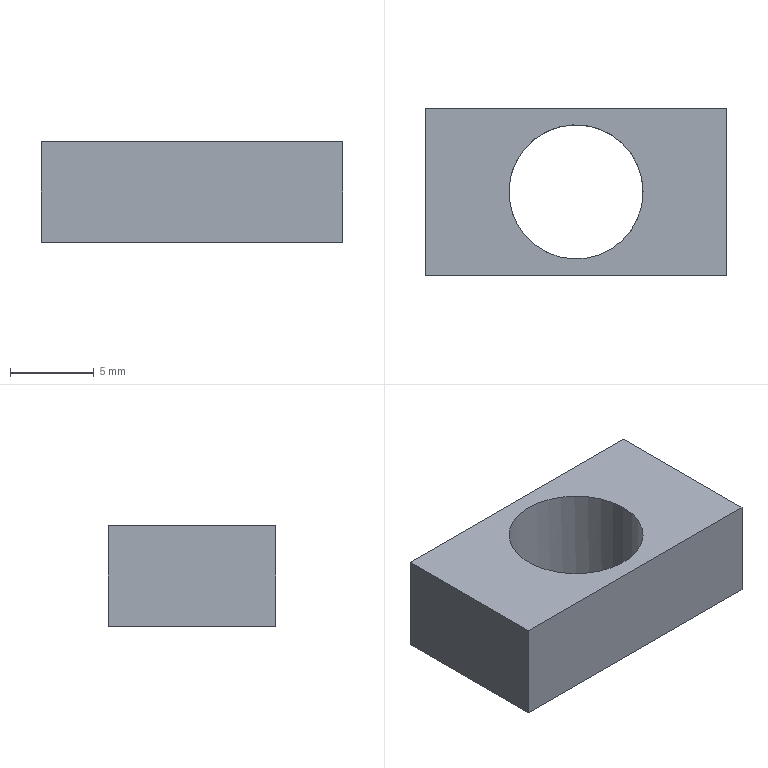Component | NX | WORKPIECE_PROCESSED | 1 solid | 7 faces | box 18 x 10 x 6 mm | volume 778 mm3 | plane 6 | cylinder 1 | commonest cylinder face diameters 8 x1
STEP:
#1=CARTESIAN_POINT('',(0.,0.,0.));
#2=DIRECTION('',(0.,0.,1.));
#3=DIRECTION('',(1.,0.,0.));
#4=AXIS2_PLACEMENT_3D('',#1,#2,#3);
#5=CARTESIAN_POINT('',(-142.329,14.498,29.));
#6=VERTEX_POINT('',#5);
#7=CARTESIAN_POINT('',(-146.329,14.498,29.));
#8=DIRECTION('',(0.,0.,1.));
#9=DIRECTION('',(1.,0.,0.));
#10=AXIS2_PLACEMENT_3D('',#7,#8,#9);
#11=CIRCLE('',#10,4.);
#12=CARTESIAN_POINT('',(-146.329,14.498,29.));
#13=DIRECTION('',(0.,0.,1.));
#14=DIRECTION('',(1.,0.,0.));
#15=AXIS2_PLACEMENT_3D('',#12,#13,#14);
#16=PLANE('',#15);
#17=CARTESIAN_POINT('',(0.,0.));
#18=DIRECTION('',(1.,0.));
#19=AXIS2_PLACEMENT_2D('',#17,#18);
#20=CIRCLE('',#19,4.);
#21=(GEOMETRIC_REPRESENTATION_CONTEXT(2)PARAMETRIC_REPRESENTATION_CONTEXT()REPRESENTATION_CONTEXT('',''));
#22=DEFINITIONAL_REPRESENTATION('',(#20),#21);
#23=PCURVE('',#16,#22);
#24=CARTESIAN_POINT('',(-146.329,14.498,19.5));
#25=DIRECTION('',(0.,0.,1.));
#26=DIRECTION('',(1.,0.,0.));
#27=AXIS2_PLACEMENT_3D('',#24,#25,#26);
#28=CYLINDRICAL_SURFACE('',#27,4.);
#29=CARTESIAN_POINT('',(0.,9.5));
#30=DIRECTION('',(1.,0.));
#31=VECTOR('',#30,1.);
#32=LINE('',#29,#31);
#33=(GEOMETRIC_REPRESENTATION_CONTEXT(2)PARAMETRIC_REPRESENTATION_CONTEXT()REPRESENTATION_CONTEXT('',''));
#34=DEFINITIONAL_REPRESENTATION('',(#32),#33);
#35=PCURVE('',#28,#34);
#36=SURFACE_CURVE('',#11,(#23,#35),.PCURVE_S1.);
#37=EDGE_CURVE('',#6,#6,#36,.T.);
#38=ORIENTED_EDGE('',*,*,#37,.F.);
#39=EDGE_LOOP('',(#38));
#40=FACE_BOUND('',#39,.T.);
#41=CARTESIAN_POINT('',(-137.329,9.498,29.));
#42=VERTEX_POINT('',#41);
#43=CARTESIAN_POINT('',(-155.329,9.498,29.));
#44=VERTEX_POINT('',#43);
#45=CARTESIAN_POINT('',(-146.329,9.498,29.));
#46=DIRECTION('',(-1.,0.,0.));
#47=VECTOR('',#46,1.);
#48=LINE('',#45,#47);
#49=CARTESIAN_POINT('',(0.,-5.));
#50=DIRECTION('',(-1.,0.));
#51=VECTOR('',#50,1.);
#52=LINE('',#49,#51);
#53=(GEOMETRIC_REPRESENTATION_CONTEXT(2)PARAMETRIC_REPRESENTATION_CONTEXT()REPRESENTATION_CONTEXT('',''));
#54=DEFINITIONAL_REPRESENTATION('',(#52),#53);
#55=PCURVE('',#16,#54);
#56=CARTESIAN_POINT('',(-146.329,9.498,23.));
#57=DIRECTION('',(0.,-1.,0.));
#58=DIRECTION('',(0.,0.,-1.));
#59=AXIS2_PLACEMENT_3D('',#56,#57,#58);
#60=PLANE('',#59);
#61=CARTESIAN_POINT('',(-6.,0.));
#62=DIRECTION('',(0.,-1.));
#63=VECTOR('',#62,1.);
#64=LINE('',#61,#63);
#65=(GEOMETRIC_REPRESENTATION_CONTEXT(2)PARAMETRIC_REPRESENTATION_CONTEXT()REPRESENTATION_CONTEXT('',''));
#66=DEFINITIONAL_REPRESENTATION('',(#64),#65);
#67=PCURVE('',#60,#66);
#68=SURFACE_CURVE('',#48,(#55,#67),.PCURVE_S1.);
#69=EDGE_CURVE('',#42,#44,#68,.T.);
#70=ORIENTED_EDGE('',*,*,#69,.F.);
#71=CARTESIAN_POINT('',(-137.329,19.498,29.));
#72=VERTEX_POINT('',#71);
#73=CARTESIAN_POINT('',(-137.329,14.498,29.));
#74=DIRECTION('',(0.,-1.,0.));
#75=VECTOR('',#74,1.);
#76=LINE('',#73,#75);
#77=CARTESIAN_POINT('',(9.,0.));
#78=DIRECTION('',(0.,-1.));
#79=VECTOR('',#78,1.);
#80=LINE('',#77,#79);
#81=(GEOMETRIC_REPRESENTATION_CONTEXT(2)PARAMETRIC_REPRESENTATION_CONTEXT()REPRESENTATION_CONTEXT('',''));
#82=DEFINITIONAL_REPRESENTATION('',(#80),#81);
#83=PCURVE('',#16,#82);
#84=CARTESIAN_POINT('',(-137.329,14.498,23.));
#85=DIRECTION('',(1.,0.,0.));
#86=DIRECTION('',(0.,0.,-1.));
#87=AXIS2_PLACEMENT_3D('',#84,#85,#86);
#88=PLANE('',#87);
#89=CARTESIAN_POINT('',(-6.,0.));
#90=DIRECTION('',(0.,-1.));
#91=VECTOR('',#90,1.);
#92=LINE('',#89,#91);
#93=(GEOMETRIC_REPRESENTATION_CONTEXT(2)PARAMETRIC_REPRESENTATION_CONTEXT()REPRESENTATION_CONTEXT('',''));
#94=DEFINITIONAL_REPRESENTATION('',(#92),#93);
#95=PCURVE('',#88,#94);
#96=SURFACE_CURVE('',#76,(#83,#95),.PCURVE_S1.);
#97=EDGE_CURVE('',#72,#42,#96,.T.);
#98=ORIENTED_EDGE('',*,*,#97,.F.);
#99=CARTESIAN_POINT('',(-155.329,19.498,29.));
#100=VERTEX_POINT('',#99);
#101=CARTESIAN_POINT('',(-146.329,19.498,29.));
#102=DIRECTION('',(1.,0.,0.));
#103=VECTOR('',#102,1.);
#104=LINE('',#101,#103);
#105=CARTESIAN_POINT('',(0.,5.));
#106=DIRECTION('',(1.,0.));
#107=VECTOR('',#106,1.);
#108=LINE('',#105,#107);
#109=(GEOMETRIC_REPRESENTATION_CONTEXT(2)PARAMETRIC_REPRESENTATION_CONTEXT()REPRESENTATION_CONTEXT('',''));
#110=DEFINITIONAL_REPRESENTATION('',(#108),#109);
#111=PCURVE('',#16,#110);
#112=CARTESIAN_POINT('',(-146.329,19.498,23.));
#113=DIRECTION('',(0.,1.,0.));
#114=DIRECTION('',(0.,0.,1.));
#115=AXIS2_PLACEMENT_3D('',#112,#113,#114);
#116=PLANE('',#115);
#117=CARTESIAN_POINT('',(6.,0.));
#118=DIRECTION('',(0.,1.));
#119=VECTOR('',#118,1.);
#120=LINE('',#117,#119);
#121=(GEOMETRIC_REPRESENTATION_CONTEXT(2)PARAMETRIC_REPRESENTATION_CONTEXT()REPRESENTATION_CONTEXT('',''));
#122=DEFINITIONAL_REPRESENTATION('',(#120),#121);
#123=PCURVE('',#116,#122);
#124=SURFACE_CURVE('',#104,(#111,#123),.PCURVE_S1.);
#125=EDGE_CURVE('',#100,#72,#124,.T.);
#126=ORIENTED_EDGE('',*,*,#125,.F.);
#127=CARTESIAN_POINT('',(-155.329,14.498,29.));
#128=DIRECTION('',(0.,1.,0.));
#129=VECTOR('',#128,1.);
#130=LINE('',#127,#129);
#131=CARTESIAN_POINT('',(-9.,0.));
#132=DIRECTION('',(0.,1.));
#133=VECTOR('',#132,1.);
#134=LINE('',#131,#133);
#135=(GEOMETRIC_REPRESENTATION_CONTEXT(2)PARAMETRIC_REPRESENTATION_CONTEXT()REPRESENTATION_CONTEXT('',''));
#136=DEFINITIONAL_REPRESENTATION('',(#134),#135);
#137=PCURVE('',#16,#136);
#138=CARTESIAN_POINT('',(-155.329,14.498,23.));
#139=DIRECTION('',(-1.,0.,0.));
#140=DIRECTION('',(0.,0.,1.));
#141=AXIS2_PLACEMENT_3D('',#138,#139,#140);
#142=PLANE('',#141);
#143=CARTESIAN_POINT('',(6.,0.));
#144=DIRECTION('',(0.,1.));
#145=VECTOR('',#144,1.);
#146=LINE('',#143,#145);
#147=(GEOMETRIC_REPRESENTATION_CONTEXT(2)PARAMETRIC_REPRESENTATION_CONTEXT()REPRESENTATION_CONTEXT('',''));
#148=DEFINITIONAL_REPRESENTATION('',(#146),#147);
#149=PCURVE('',#142,#148);
#150=SURFACE_CURVE('',#130,(#137,#149),.PCURVE_S1.);
#151=EDGE_CURVE('',#44,#100,#150,.T.);
#152=ORIENTED_EDGE('',*,*,#151,.F.);
#153=EDGE_LOOP('',(#70,#98,#126,#152));
#154=FACE_BOUND('',#153,.T.);
#155=ADVANCED_FACE('',(#40,#154),#16,.T.);
#156=CARTESIAN_POINT('',(-137.329,9.498,23.));
#157=VERTEX_POINT('',#156);
#158=CARTESIAN_POINT('',(-137.329,9.498,23.));
#159=DIRECTION('',(0.,0.,1.));
#160=VECTOR('',#159,1.);
#161=LINE('',#158,#160);
#162=CARTESIAN_POINT('',(0.,9.));
#163=DIRECTION('',(-1.,0.));
#164=VECTOR('',#163,1.);
#165=LINE('',#162,#164);
#166=(GEOMETRIC_REPRESENTATION_CONTEXT(2)PARAMETRIC_REPRESENTATION_CONTEXT()REPRESENTATION_CONTEXT('',''));
#167=DEFINITIONAL_REPRESENTATION('',(#165),#166);
#168=PCURVE('',#60,#167);
#169=CARTESIAN_POINT('',(0.,-5.));
#170=DIRECTION('',(-1.,0.));
#171=VECTOR('',#170,1.);
#172=LINE('',#169,#171);
#173=(GEOMETRIC_REPRESENTATION_CONTEXT(2)PARAMETRIC_REPRESENTATION_CONTEXT()REPRESENTATION_CONTEXT('',''));
#174=DEFINITIONAL_REPRESENTATION('',(#172),#173);
#175=PCURVE('',#88,#174);
#176=SURFACE_CURVE('',#161,(#168,#175),.PCURVE_S1.);
#177=EDGE_CURVE('',#157,#42,#176,.T.);
#178=ORIENTED_EDGE('',*,*,#177,.T.);
#179=ORIENTED_EDGE('',*,*,#69,.T.);
#180=CARTESIAN_POINT('',(-155.329,9.498,23.));
#181=VERTEX_POINT('',#180);
#182=CARTESIAN_POINT('',(-155.329,9.498,23.));
#183=DIRECTION('',(0.,0.,1.));
#184=VECTOR('',#183,1.);
#185=LINE('',#182,#184);
#186=CARTESIAN_POINT('',(0.,-9.));
#187=DIRECTION('',(-1.,0.));
#188=VECTOR('',#187,1.);
#189=LINE('',#186,#188);
#190=(GEOMETRIC_REPRESENTATION_CONTEXT(2)PARAMETRIC_REPRESENTATION_CONTEXT()REPRESENTATION_CONTEXT('',''));
#191=DEFINITIONAL_REPRESENTATION('',(#189),#190);
#192=PCURVE('',#60,#191);
#193=CARTESIAN_POINT('',(0.,-5.));
#194=DIRECTION('',(1.,0.));
#195=VECTOR('',#194,1.);
#196=LINE('',#193,#195);
#197=(GEOMETRIC_REPRESENTATION_CONTEXT(2)PARAMETRIC_REPRESENTATION_CONTEXT()REPRESENTATION_CONTEXT('',''));
#198=DEFINITIONAL_REPRESENTATION('',(#196),#197);
#199=PCURVE('',#142,#198);
#200=SURFACE_CURVE('',#185,(#192,#199),.PCURVE_S1.);
#201=EDGE_CURVE('',#181,#44,#200,.T.);
#202=ORIENTED_EDGE('',*,*,#201,.F.);
#203=CARTESIAN_POINT('',(-146.329,9.498,23.));
#204=DIRECTION('',(1.,0.,0.));
#205=VECTOR('',#204,1.);
#206=LINE('',#203,#205);
#207=CARTESIAN_POINT('',(0.,0.));
#208=DIRECTION('',(0.,1.));
#209=VECTOR('',#208,1.);
#210=LINE('',#207,#209);
#211=(GEOMETRIC_REPRESENTATION_CONTEXT(2)PARAMETRIC_REPRESENTATION_CONTEXT()REPRESENTATION_CONTEXT('',''));
#212=DEFINITIONAL_REPRESENTATION('',(#210),#211);
#213=PCURVE('',#60,#212);
#214=CARTESIAN_POINT('',(-146.329,14.498,23.));
#215=DIRECTION('',(0.,0.,-1.));
#216=DIRECTION('',(-1.,0.,0.));
#217=AXIS2_PLACEMENT_3D('',#214,#215,#216);
#218=PLANE('',#217);
#219=CARTESIAN_POINT('',(0.,-5.));
#220=DIRECTION('',(-1.,0.));
#221=VECTOR('',#220,1.);
#222=LINE('',#219,#221);
#223=(GEOMETRIC_REPRESENTATION_CONTEXT(2)PARAMETRIC_REPRESENTATION_CONTEXT()REPRESENTATION_CONTEXT('',''));
#224=DEFINITIONAL_REPRESENTATION('',(#222),#223);
#225=PCURVE('',#218,#224);
#226=SURFACE_CURVE('',#206,(#213,#225),.PCURVE_S1.);
#227=EDGE_CURVE('',#181,#157,#226,.T.);
#228=ORIENTED_EDGE('',*,*,#227,.T.);
#229=EDGE_LOOP('',(#178,#179,#202,#228));
#230=FACE_BOUND('',#229,.T.);
#231=ADVANCED_FACE('',(#230),#60,.T.);
#232=ORIENTED_EDGE('',*,*,#201,.T.);
#233=ORIENTED_EDGE('',*,*,#151,.T.);
#234=CARTESIAN_POINT('',(-155.329,19.498,23.));
#235=VERTEX_POINT('',#234);
#236=CARTESIAN_POINT('',(-155.329,19.498,23.));
#237=DIRECTION('',(0.,0.,1.));
#238=VECTOR('',#237,1.);
#239=LINE('',#236,#238);
#240=CARTESIAN_POINT('',(0.,5.));
#241=DIRECTION('',(1.,0.));
#242=VECTOR('',#241,1.);
#243=LINE('',#240,#242);
#244=(GEOMETRIC_REPRESENTATION_CONTEXT(2)PARAMETRIC_REPRESENTATION_CONTEXT()REPRESENTATION_CONTEXT('',''));
#245=DEFINITIONAL_REPRESENTATION('',(#243),#244);
#246=PCURVE('',#142,#245);
#247=CARTESIAN_POINT('',(0.,-9.));
#248=DIRECTION('',(1.,0.));
#249=VECTOR('',#248,1.);
#250=LINE('',#247,#249);
#251=(GEOMETRIC_REPRESENTATION_CONTEXT(2)PARAMETRIC_REPRESENTATION_CONTEXT()REPRESENTATION_CONTEXT('',''));
#252=DEFINITIONAL_REPRESENTATION('',(#250),#251);
#253=PCURVE('',#116,#252);
#254=SURFACE_CURVE('',#239,(#246,#253),.PCURVE_S1.);
#255=EDGE_CURVE('',#235,#100,#254,.T.);
#256=ORIENTED_EDGE('',*,*,#255,.F.);
#257=CARTESIAN_POINT('',(-155.329,14.498,23.));
#258=DIRECTION('',(0.,-1.,0.));
#259=VECTOR('',#258,1.);
#260=LINE('',#257,#259);
#261=CARTESIAN_POINT('',(0.,0.));
#262=DIRECTION('',(0.,-1.));
#263=VECTOR('',#262,1.);
#264=LINE('',#261,#263);
#265=(GEOMETRIC_REPRESENTATION_CONTEXT(2)PARAMETRIC_REPRESENTATION_CONTEXT()REPRESENTATION_CONTEXT('',''));
#266=DEFINITIONAL_REPRESENTATION('',(#264),#265);
#267=PCURVE('',#142,#266);
#268=CARTESIAN_POINT('',(9.,0.));
#269=DIRECTION('',(0.,-1.));
#270=VECTOR('',#269,1.);
#271=LINE('',#268,#270);
#272=(GEOMETRIC_REPRESENTATION_CONTEXT(2)PARAMETRIC_REPRESENTATION_CONTEXT()REPRESENTATION_CONTEXT('',''));
#273=DEFINITIONAL_REPRESENTATION('',(#271),#272);
#274=PCURVE('',#218,#273);
#275=SURFACE_CURVE('',#260,(#267,#274),.PCURVE_S1.);
#276=EDGE_CURVE('',#235,#181,#275,.T.);
#277=ORIENTED_EDGE('',*,*,#276,.T.);
#278=EDGE_LOOP('',(#232,#233,#256,#277));
#279=FACE_BOUND('',#278,.T.);
#280=ADVANCED_FACE('',(#279),#142,.T.);
#281=ORIENTED_EDGE('',*,*,#255,.T.);
#282=ORIENTED_EDGE('',*,*,#125,.T.);
#283=CARTESIAN_POINT('',(-137.329,19.498,23.));
#284=VERTEX_POINT('',#283);
#285=CARTESIAN_POINT('',(-137.329,19.498,23.));
#286=DIRECTION('',(0.,0.,1.));
#287=VECTOR('',#286,1.);
#288=LINE('',#285,#287);
#289=CARTESIAN_POINT('',(0.,9.));
#290=DIRECTION('',(1.,0.));
#291=VECTOR('',#290,1.);
#292=LINE('',#289,#291);
#293=(GEOMETRIC_REPRESENTATION_CONTEXT(2)PARAMETRIC_REPRESENTATION_CONTEXT()REPRESENTATION_CONTEXT('',''));
#294=DEFINITIONAL_REPRESENTATION('',(#292),#293);
#295=PCURVE('',#116,#294);
#296=CARTESIAN_POINT('',(0.,5.));
#297=DIRECTION('',(-1.,0.));
#298=VECTOR('',#297,1.);
#299=LINE('',#296,#298);
#300=(GEOMETRIC_REPRESENTATION_CONTEXT(2)PARAMETRIC_REPRESENTATION_CONTEXT()REPRESENTATION_CONTEXT('',''));
#301=DEFINITIONAL_REPRESENTATION('',(#299),#300);
#302=PCURVE('',#88,#301);
#303=SURFACE_CURVE('',#288,(#295,#302),.PCURVE_S1.);
#304=EDGE_CURVE('',#284,#72,#303,.T.);
#305=ORIENTED_EDGE('',*,*,#304,.F.);
#306=CARTESIAN_POINT('',(-146.329,19.498,23.));
#307=DIRECTION('',(-1.,0.,0.));
#308=VECTOR('',#307,1.);
#309=LINE('',#306,#308);
#310=CARTESIAN_POINT('',(0.,0.));
#311=DIRECTION('',(0.,-1.));
#312=VECTOR('',#311,1.);
#313=LINE('',#310,#312);
#314=(GEOMETRIC_REPRESENTATION_CONTEXT(2)PARAMETRIC_REPRESENTATION_CONTEXT()REPRESENTATION_CONTEXT('',''));
#315=DEFINITIONAL_REPRESENTATION('',(#313),#314);
#316=PCURVE('',#116,#315);
#317=CARTESIAN_POINT('',(0.,5.));
#318=DIRECTION('',(1.,0.));
#319=VECTOR('',#318,1.);
#320=LINE('',#317,#319);
#321=(GEOMETRIC_REPRESENTATION_CONTEXT(2)PARAMETRIC_REPRESENTATION_CONTEXT()REPRESENTATION_CONTEXT('',''));
#322=DEFINITIONAL_REPRESENTATION('',(#320),#321);
#323=PCURVE('',#218,#322);
#324=SURFACE_CURVE('',#309,(#316,#323),.PCURVE_S1.);
#325=EDGE_CURVE('',#284,#235,#324,.T.);
#326=ORIENTED_EDGE('',*,*,#325,.T.);
#327=EDGE_LOOP('',(#281,#282,#305,#326));
#328=FACE_BOUND('',#327,.T.);
#329=ADVANCED_FACE('',(#328),#116,.T.);
#330=CARTESIAN_POINT('',(-150.329,14.498,23.));
#331=VERTEX_POINT('',#330);
#332=CARTESIAN_POINT('',(-142.329,14.498,23.));
#333=VERTEX_POINT('',#332);
#334=CARTESIAN_POINT('',(-146.329,14.498,23.));
#335=DIRECTION('',(0.,0.,-1.));
#336=DIRECTION('',(-1.,0.,0.));
#337=AXIS2_PLACEMENT_3D('',#334,#335,#336);
#338=CIRCLE('',#337,4.);
#339=CARTESIAN_POINT('',(0.,0.));
#340=DIRECTION('',(1.,0.));
#341=AXIS2_PLACEMENT_2D('',#339,#340);
#342=CIRCLE('',#341,4.);
#343=(GEOMETRIC_REPRESENTATION_CONTEXT(2)PARAMETRIC_REPRESENTATION_CONTEXT()REPRESENTATION_CONTEXT('',''));
#344=DEFINITIONAL_REPRESENTATION('',(#342),#343);
#345=PCURVE('',#218,#344);
#346=CARTESIAN_POINT('',(3.142,3.5));
#347=DIRECTION('',(-1.,0.));
#348=VECTOR('',#347,1.);
#349=LINE('',#346,#348);
#350=(GEOMETRIC_REPRESENTATION_CONTEXT(2)PARAMETRIC_REPRESENTATION_CONTEXT()REPRESENTATION_CONTEXT('',''));
#351=DEFINITIONAL_REPRESENTATION('',(#349),#350);
#352=PCURVE('',#28,#351);
#353=SURFACE_CURVE('',#338,(#345,#352),.PCURVE_S1.);
#354=EDGE_CURVE('',#331,#333,#353,.T.);
#355=ORIENTED_EDGE('',*,*,#354,.F.);
#356=CARTESIAN_POINT('',(-146.329,14.498,23.));
#357=DIRECTION('',(0.,0.,-1.));
#358=DIRECTION('',(-1.,0.,0.));
#359=AXIS2_PLACEMENT_3D('',#356,#357,#358);
#360=CIRCLE('',#359,4.);
#361=CARTESIAN_POINT('',(0.,0.));
#362=DIRECTION('',(1.,0.));
#363=AXIS2_PLACEMENT_2D('',#361,#362);
#364=CIRCLE('',#363,4.);
#365=(GEOMETRIC_REPRESENTATION_CONTEXT(2)PARAMETRIC_REPRESENTATION_CONTEXT()REPRESENTATION_CONTEXT('',''));
#366=DEFINITIONAL_REPRESENTATION('',(#364),#365);
#367=PCURVE('',#218,#366);
#368=CARTESIAN_POINT('',(9.425,3.5));
#369=DIRECTION('',(-1.,0.));
#370=VECTOR('',#369,1.);
#371=LINE('',#368,#370);
#372=(GEOMETRIC_REPRESENTATION_CONTEXT(2)PARAMETRIC_REPRESENTATION_CONTEXT()REPRESENTATION_CONTEXT('',''));
#373=DEFINITIONAL_REPRESENTATION('',(#371),#372);
#374=PCURVE('',#28,#373);
#375=SURFACE_CURVE('',#360,(#367,#374),.PCURVE_S1.);
#376=EDGE_CURVE('',#333,#331,#375,.T.);
#377=ORIENTED_EDGE('',*,*,#376,.F.);
#378=EDGE_LOOP('',(#355,#377));
#379=FACE_BOUND('',#378,.T.);
#380=CARTESIAN_POINT('',(-137.329,14.498,23.));
#381=DIRECTION('',(0.,1.,0.));
#382=VECTOR('',#381,1.);
#383=LINE('',#380,#382);
#384=CARTESIAN_POINT('',(-9.,0.));
#385=DIRECTION('',(0.,1.));
#386=VECTOR('',#385,1.);
#387=LINE('',#384,#386);
#388=(GEOMETRIC_REPRESENTATION_CONTEXT(2)PARAMETRIC_REPRESENTATION_CONTEXT()REPRESENTATION_CONTEXT('',''));
#389=DEFINITIONAL_REPRESENTATION('',(#387),#388);
#390=PCURVE('',#218,#389);
#391=CARTESIAN_POINT('',(0.,0.));
#392=DIRECTION('',(0.,1.));
#393=VECTOR('',#392,1.);
#394=LINE('',#391,#393);
#395=(GEOMETRIC_REPRESENTATION_CONTEXT(2)PARAMETRIC_REPRESENTATION_CONTEXT()REPRESENTATION_CONTEXT('',''));
#396=DEFINITIONAL_REPRESENTATION('',(#394),#395);
#397=PCURVE('',#88,#396);
#398=SURFACE_CURVE('',#383,(#390,#397),.PCURVE_S1.);
#399=EDGE_CURVE('',#157,#284,#398,.T.);
#400=ORIENTED_EDGE('',*,*,#399,.F.);
#401=ORIENTED_EDGE('',*,*,#227,.F.);
#402=ORIENTED_EDGE('',*,*,#276,.F.);
#403=ORIENTED_EDGE('',*,*,#325,.F.);
#404=EDGE_LOOP('',(#400,#401,#402,#403));
#405=FACE_BOUND('',#404,.T.);
#406=ADVANCED_FACE('',(#379,#405),#218,.T.);
#407=ORIENTED_EDGE('',*,*,#399,.T.);
#408=ORIENTED_EDGE('',*,*,#304,.T.);
#409=ORIENTED_EDGE('',*,*,#97,.T.);
#410=ORIENTED_EDGE('',*,*,#177,.F.);
#411=EDGE_LOOP('',(#407,#408,#409,#410));
#412=FACE_BOUND('',#411,.T.);
#413=ADVANCED_FACE('',(#412),#88,.T.);
#414=ORIENTED_EDGE('',*,*,#376,.F.);
#415=CARTESIAN_POINT('',(-142.329,14.498,23.));
#416=CARTESIAN_POINT('',(-142.329,14.498,29.));
#417=B_SPLINE_CURVE_WITH_KNOTS('',1,(#415,#416),.UNSPECIFIED.,.F.,.F.,(2,2),(3.5,9.5),.PIECEWISE_BEZIER_KNOTS.);
#418=CARTESIAN_POINT('',(6.283,0.));
#419=DIRECTION('',(0.,1.));
#420=VECTOR('',#419,1.);
#421=LINE('',#418,#420);
#422=(GEOMETRIC_REPRESENTATION_CONTEXT(2)PARAMETRIC_REPRESENTATION_CONTEXT()REPRESENTATION_CONTEXT('',''));
#423=DEFINITIONAL_REPRESENTATION('',(#421),#422);
#424=PCURVE('',#28,#423);
#425=CARTESIAN_POINT('',(0.,0.));
#426=DIRECTION('',(0.,1.));
#427=VECTOR('',#426,1.);
#428=LINE('',#425,#427);
#429=(GEOMETRIC_REPRESENTATION_CONTEXT(2)PARAMETRIC_REPRESENTATION_CONTEXT()REPRESENTATION_CONTEXT('',''));
#430=DEFINITIONAL_REPRESENTATION('',(#428),#429);
#431=PCURVE('',#28,#430);
#432=SEAM_CURVE('',#417,(#424,#431),.PCURVE_S1.);
#433=EDGE_CURVE('',#333,#6,#432,.T.);
#434=ORIENTED_EDGE('',*,*,#433,.T.);
#435=ORIENTED_EDGE('',*,*,#37,.F.);
#436=ORIENTED_EDGE('',*,*,#433,.F.);
#437=ORIENTED_EDGE('',*,*,#354,.F.);
#438=EDGE_LOOP('',(#414,#434,#435,#436,#437));
#439=FACE_BOUND('',#438,.F.);
#440=ADVANCED_FACE('',(#439),#28,.F.);
#441=CLOSED_SHELL('',(#155,#231,#280,#329,#406,#413,#440));
#442=MANIFOLD_SOLID_BREP('',#441);
#443=(LENGTH_UNIT()NAMED_UNIT(*)SI_UNIT(.MILLI.,.METRE.));
#444=UNCERTAINTY_MEASURE_WITH_UNIT(LENGTH_MEASURE(0.000002),#443,'','');
#445=(NAMED_UNIT(*)PLANE_ANGLE_UNIT()SI_UNIT($,.RADIAN.));
#446=(NAMED_UNIT(*)SI_UNIT($,.STERADIAN.)SOLID_ANGLE_UNIT());
#447=(GEOMETRIC_REPRESENTATION_CONTEXT(3)GLOBAL_UNCERTAINTY_ASSIGNED_CONTEXT((#444))GLOBAL_UNIT_ASSIGNED_CONTEXT((#443,#445,#446))REPRESENTATION_CONTEXT('',''));
#448=ADVANCED_BREP_SHAPE_REPRESENTATION('',(#4,#442),#447);